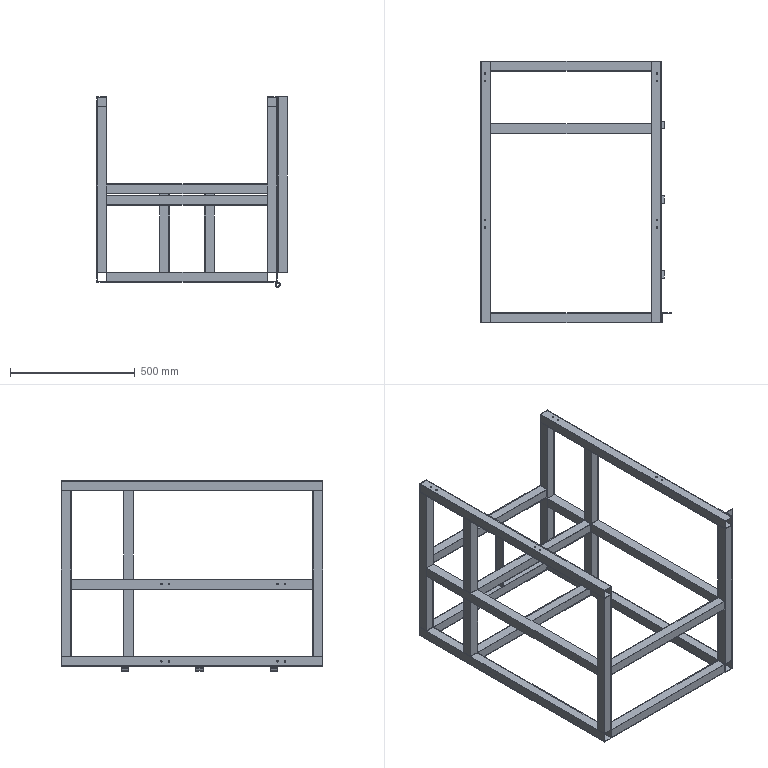Component | SolidWorks | FrameAssembly-1_FrameWeldment-1_Frame-1 | 25 solids | 296 faces | volume 6200391 mm3 | plane 250 | cylinder 46 | commonest cylinder face diameters 6 x32 9 x8 20 x3 12 x3